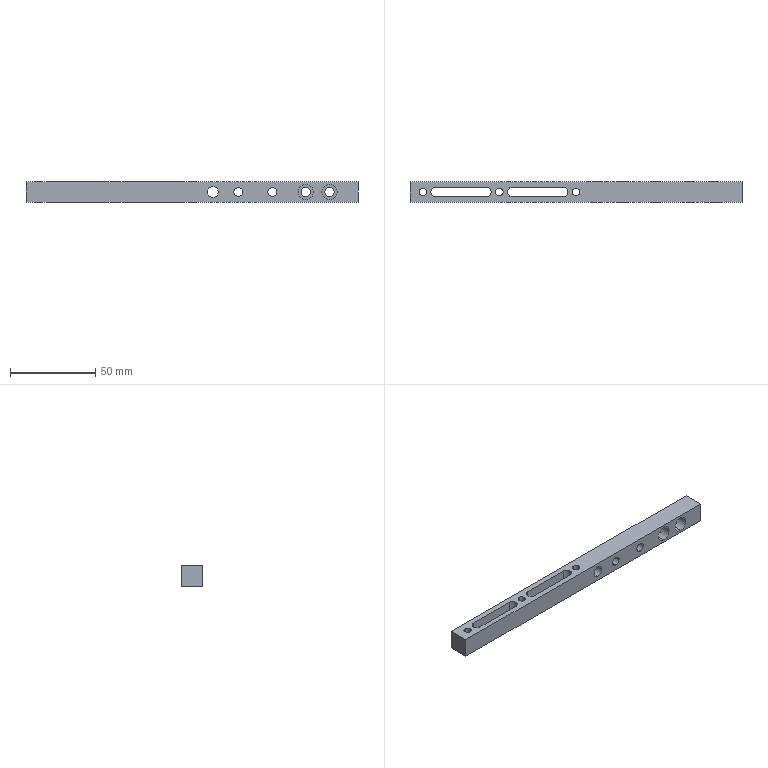CAM job | Mastercam | mm | 8 operations | part box 195 x 12 x 12
1. Drill/Counterbore | 2 - 6 定位钻
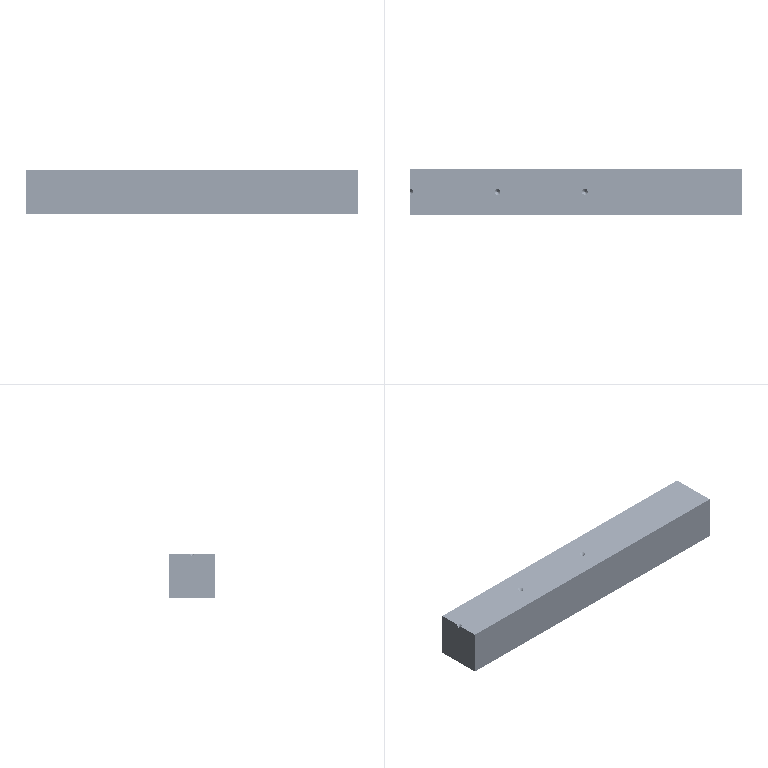2. Peck Drill | 20 - 4.3 钻头
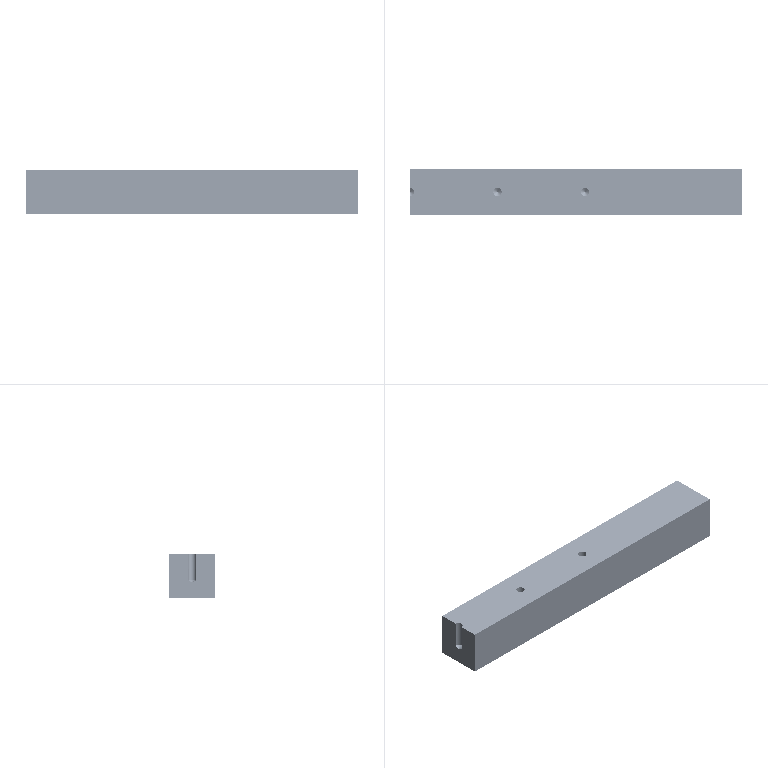3. Contour (Ramp) | 3 - 5 平铣刀
4. Drill/Counterbore | 2 - 6 定位钻
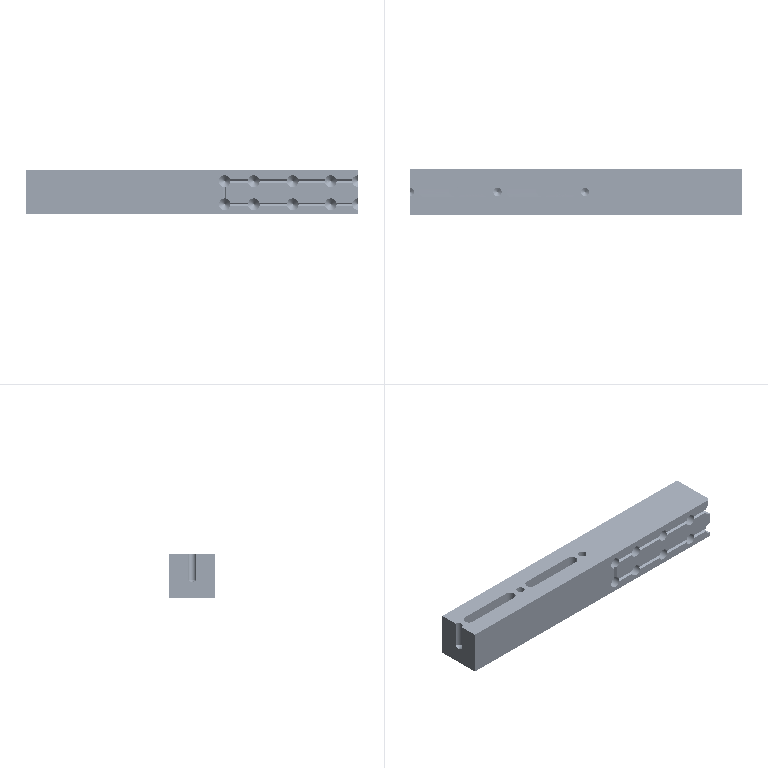5. Peck Drill | 1 - 5.3 钻头
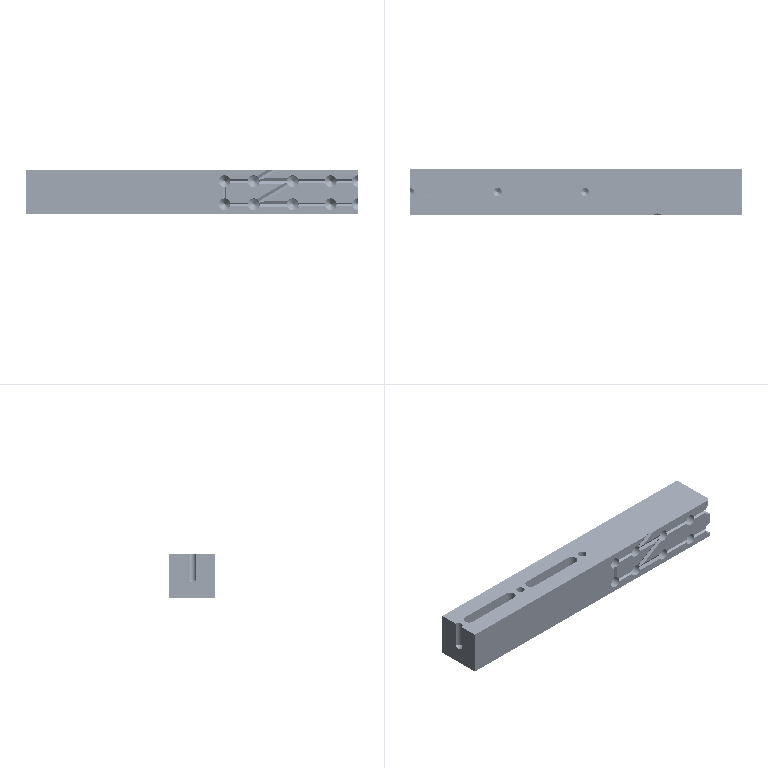6. Peck Drill | 16 - 5.5 钻头
7. Peck Drill | 15 - 9 平铣刀
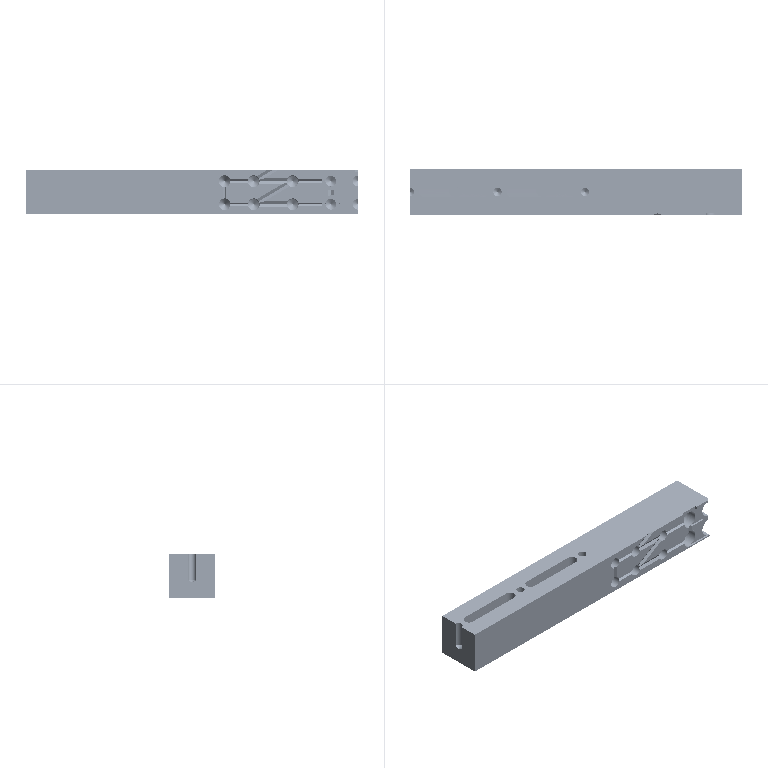8. Peck Drill | 20 - 6.5 钻头